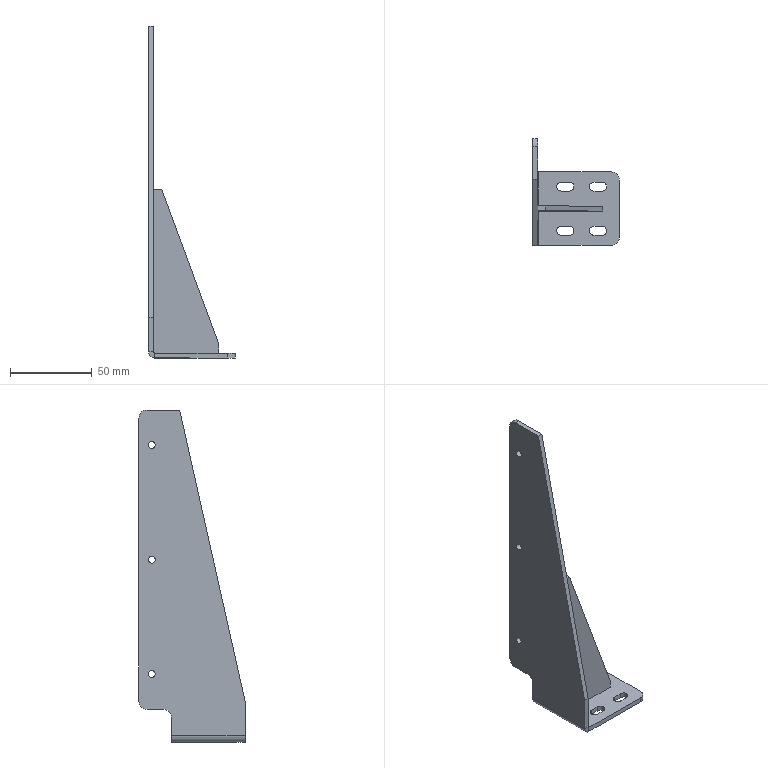Component | SolidWorks | 01-16ElectricalControlPanelBracket-1 | 1 solid | 52 faces | volume 40549 mm3 | cylinder 26 | plane 26 | commonest cylinder face diameters 5.5 x12 4.2 x6 10 x5 1.473 x2 7.473 x1 | material SGLCC